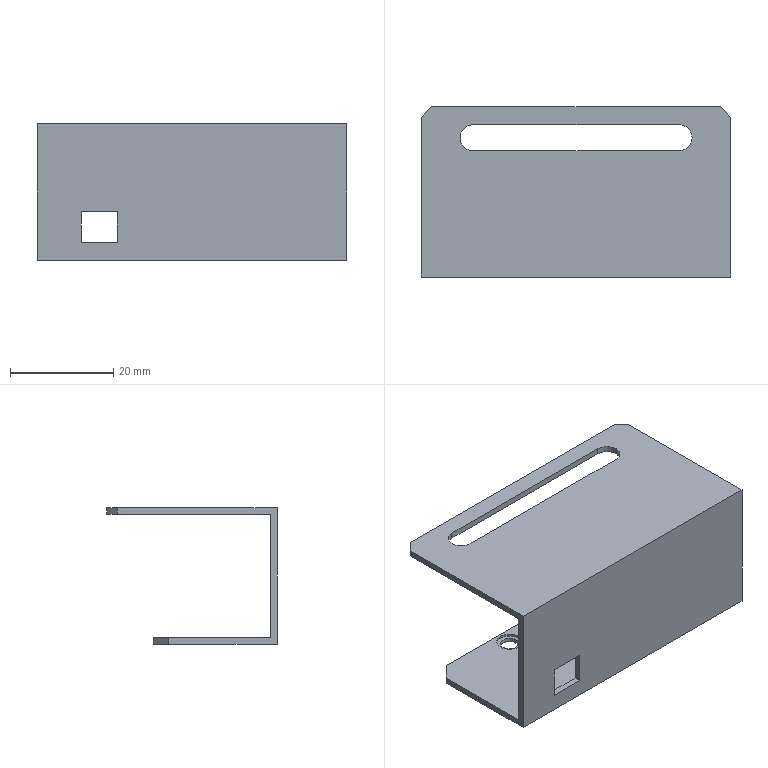Component | SolidWorks | SL010-RightStreamline-1-1_SL010-SensorAssembly-F-1-2_SL010-0ALk-010000-012-2-1-1 | 1 solid | 33 faces | box 60 x 33 x 26.4 mm | volume 5471 mm3 | plane 22 | cylinder 11 | commonest cylinder face diameters 5 x7 3.5 x4 | material 304
build123d program:
from build123d import *

# Parameters (mm, degrees)
SKETCH1_2_W                    = 60
SKETCH1_2_H                    = 33
BOSS_EXTRUDE1_DEPTH            = 1.2
CUT_EXTRUDE1_2_DEPTH           = 35.259
CHAMFER2_SIZE                  = 2
SKETCH6_W                      = 60
SKETCH6_H                      = 1.2
BOSS_EXTRUDE2_DEPTH            = 24
SKETCH7_W                      = 60
SKETCH7_H                      = 24
BOSS_EXTRUDE3_DEPTH            = 1.2
CHAMFER3_SIZE                  = 3
F_3_5_3_5_DIAMETER_HOLE1_D     = 3.5
F_3_5_3_5_DIAMETER_HOLE1_DEPTH = 1.2
SKETCH1_W                      = 7
SKETCH1_H                      = 6
CUT_EXTRUDE1_DEPTH             = 52.071
SKETCH2_R                      = 2.5
CUT_EXTRUDE2_DEPTH             = 0.4


with BuildPart() as part:
    # Sketch1_2 → Boss-Extrude1 (new body)
    with BuildSketch(Plane.XY):
        Rectangle(SKETCH1_2_W, SKETCH1_2_H)
    extrude(amount=BOSS_EXTRUDE1_DEPTH)

    # Sketch2_2 → Cut-Extrude1_2 (cut, through all)
    with BuildSketch(Plane(origin=(0, 0, 0), x_dir=(-1, 0, 0), z_dir=(0, 0, -1))):
        with BuildLine():
            Line((-20, 13), (10, 13))
            ThreePointArc((10, 13), (12.5, 10.5), (10, 8))
            Line((10, 8), (-20, 8))
            ThreePointArc((-20, 8), (-22.5, 10.5), (-20, 13))
        make_face()
    cut_extrude1_2 = extrude(amount=-CUT_EXTRUDE1_2_DEPTH, mode=Mode.SUBTRACT)

    # Mirror1: Cut-Extrude1_2 across plane
    add(cut_extrude1_2.mirror(Plane(origin=(0, 0, 0), x_dir=(0, 0, 1), z_dir=(1, 0, 0))), mode=Mode.SUBTRACT)

    # Chamfer2
    chamfer2_edges = [part.edges().sort_by_distance(p)[0] for p in [
        (-30, 16.5, 0.6),
        (30, 16.5, 0.6),
    ]]
    chamfer(chamfer2_edges, length=CHAMFER2_SIZE)

    # Sketch6 → Boss-Extrude2 (add)
    with BuildSketch(Plane.XY.offset(1.2)):
        with Locations((0, -15.9)):
            Rectangle(SKETCH6_W, SKETCH6_H)
    extrude(amount=BOSS_EXTRUDE2_DEPTH)

    # Sketch7 → Boss-Extrude3 (add)
    with BuildSketch(Plane.XY.offset(25.2)):
        with Locations((0, -4.5)):
            Rectangle(SKETCH7_W, SKETCH7_H)
    extrude(amount=BOSS_EXTRUDE3_DEPTH)

    # Chamfer3
    chamfer3_edges = [part.edges().sort_by_distance(p)[0] for p in [
        (-30, 7.5, 25.8),
        (30, 7.5, 25.8),
    ]]
    chamfer(chamfer3_edges, length=CHAMFER3_SIZE)

    # 3.5 _3.5_ Diameter Hole1
    with Locations(Plane.XY.offset(26.4)):
        with Locations((12.7, 4.5), (-12.7, 4.5)):
            Hole(F_3_5_3_5_DIAMETER_HOLE1_D / 2, depth=F_3_5_3_5_DIAMETER_HOLE1_DEPTH)

    # Sketch1 → Cut-Extrude1 (cut, through all)
    with BuildSketch(Plane(origin=(0, -15.3, 0), x_dir=(1, 0, 0), z_dir=(0, 1, 0))):
        with Locations((18, -20)):
            Rectangle(SKETCH1_W, SKETCH1_H)
    extrude(amount=-CUT_EXTRUDE1_DEPTH, mode=Mode.SUBTRACT)

    # Sketch2 → Cut-Extrude2 (cut)
    with BuildSketch(Plane(origin=(0, 0, 25.2), x_dir=(-1, 0, 0), z_dir=(0, 0, -1))):
        with Locations((-12.7, 4.5)):
            Circle(SKETCH2_R)
        with Locations((12.7, 4.5)):
            Circle(SKETCH2_R)
    extrude(amount=-CUT_EXTRUDE2_DEPTH, mode=Mode.SUBTRACT)


solid = part.part

# Placed as in the assembly
solid = solid.moved(Location((355, -159.904, -331.035), (-180, 0, 180)))
STEP:
#1=COLOUR_RGB('',0.7922,0.8196,0.9333);
#2=FILL_AREA_STYLE_COLOUR('',#1);
#3=FILL_AREA_STYLE('',(#2));
#4=SURFACE_STYLE_FILL_AREA(#3);
#5=SURFACE_SIDE_STYLE('',(#4));
#6=SURFACE_STYLE_USAGE(.BOTH.,#5);
#7=PRESENTATION_STYLE_ASSIGNMENT((#6));
#8=CARTESIAN_POINT('',(14.378,-6.118,-14.041));
#9=VERTEX_POINT('',#8);
#10=CARTESIAN_POINT('',(14.575,-6.118,-14.041));
#11=VERTEX_POINT('',#10);
#12=CARTESIAN_POINT('',(14.476,-6.118,-14.041));
#13=DIRECTION('',(0.,0.,1.));
#14=DIRECTION('',(1.,0.,0.));
#15=AXIS2_PLACEMENT_3D('',#12,#13,#14);
#16=CIRCLE('',#15,0.09843);
#17=EDGE_CURVE('',#9,#11,#16,.T.);
#18=ORIENTED_EDGE('',*,*,#17,.F.);
#19=CARTESIAN_POINT('',(14.378,-6.118,-14.025));
#20=VERTEX_POINT('',#19);
#21=CARTESIAN_POINT('',(14.378,-6.118,-14.041));
#22=DIRECTION('',(0.,0.,1.));
#23=VECTOR('',#22,39.37);
#24=LINE('',#21,#23);
#25=EDGE_CURVE('',#9,#20,#24,.T.);
#26=ORIENTED_EDGE('',*,*,#25,.T.);
#27=CARTESIAN_POINT('',(14.575,-6.118,-14.025));
#28=VERTEX_POINT('',#27);
#29=CARTESIAN_POINT('',(14.476,-6.118,-14.025));
#30=DIRECTION('',(0.,0.,1.));
#31=DIRECTION('',(1.,0.,0.));
#32=AXIS2_PLACEMENT_3D('',#29,#30,#31);
#33=CIRCLE('',#32,0.09843);
#34=EDGE_CURVE('',#20,#28,#33,.T.);
#35=ORIENTED_EDGE('',*,*,#34,.T.);
#36=CARTESIAN_POINT('',(14.575,-6.118,-14.041));
#37=DIRECTION('',(0.,0.,1.));
#38=VECTOR('',#37,39.37);
#39=LINE('',#36,#38);
#40=EDGE_CURVE('',#11,#28,#39,.T.);
#41=ORIENTED_EDGE('',*,*,#40,.F.);
#42=EDGE_LOOP('',(#18,#26,#35,#41));
#43=FACE_OUTER_BOUND('',#42,.T.);
#44=CARTESIAN_POINT('',(14.476,-6.118,-14.041));
#45=DIRECTION('',(0.,0.,1.));
#46=DIRECTION('',(1.,0.,0.));
#47=AXIS2_PLACEMENT_3D('',#44,#45,#46);
#48=CYLINDRICAL_SURFACE('',#47,0.09843);
#49=ADVANCED_FACE('',(#43),#48,.F.);
#50=CARTESIAN_POINT('',(13.378,-6.118,-14.041));
#51=VERTEX_POINT('',#50);
#52=CARTESIAN_POINT('',(13.575,-6.118,-14.041));
#53=VERTEX_POINT('',#52);
#54=CARTESIAN_POINT('',(13.476,-6.118,-14.041));
#55=DIRECTION('',(0.,0.,1.));
#56=DIRECTION('',(1.,0.,0.));
#57=AXIS2_PLACEMENT_3D('',#54,#55,#56);
#58=CIRCLE('',#57,0.09843);
#59=EDGE_CURVE('',#51,#53,#58,.T.);
#60=ORIENTED_EDGE('',*,*,#59,.F.);
#61=CARTESIAN_POINT('',(13.378,-6.118,-14.025));
#62=VERTEX_POINT('',#61);
#63=CARTESIAN_POINT('',(13.378,-6.118,-14.041));
#64=DIRECTION('',(0.,0.,1.));
#65=VECTOR('',#64,39.37);
#66=LINE('',#63,#65);
#67=EDGE_CURVE('',#51,#62,#66,.T.);
#68=ORIENTED_EDGE('',*,*,#67,.T.);
#69=CARTESIAN_POINT('',(13.575,-6.118,-14.025));
#70=VERTEX_POINT('',#69);
#71=CARTESIAN_POINT('',(13.476,-6.118,-14.025));
#72=DIRECTION('',(0.,0.,1.));
#73=DIRECTION('',(1.,0.,0.));
#74=AXIS2_PLACEMENT_3D('',#71,#72,#73);
#75=CIRCLE('',#74,0.09843);
#76=EDGE_CURVE('',#62,#70,#75,.T.);
#77=ORIENTED_EDGE('',*,*,#76,.T.);
#78=CARTESIAN_POINT('',(13.575,-6.118,-14.041));
#79=DIRECTION('',(0.,0.,1.));
#80=VECTOR('',#79,39.37);
#81=LINE('',#78,#80);
#82=EDGE_CURVE('',#53,#70,#81,.T.);
#83=ORIENTED_EDGE('',*,*,#82,.F.);
#84=EDGE_LOOP('',(#60,#68,#77,#83));
#85=FACE_OUTER_BOUND('',#84,.T.);
#86=CARTESIAN_POINT('',(13.476,-6.118,-14.041));
#87=DIRECTION('',(0.,0.,1.));
#88=DIRECTION('',(1.,0.,0.));
#89=AXIS2_PLACEMENT_3D('',#86,#87,#88);
#90=CYLINDRICAL_SURFACE('',#89,0.09843);
#91=ADVANCED_FACE('',(#85),#90,.F.);
#92=CARTESIAN_POINT('',(14.764,-5.784,-13.08));
#93=VERTEX_POINT('',#92);
#94=CARTESIAN_POINT('',(14.862,-5.882,-13.08));
#95=VERTEX_POINT('',#94);
#96=CARTESIAN_POINT('',(14.764,-5.882,-13.08));
#97=DIRECTION('',(-0.,-0.,-1.));
#98=DIRECTION('',(-1.,0.,0.));
#99=AXIS2_PLACEMENT_3D('',#96,#97,#98);
#100=CIRCLE('',#99,0.09843);
#101=EDGE_CURVE('',#93,#95,#100,.T.);
#102=ORIENTED_EDGE('',*,*,#101,.T.);
#103=CARTESIAN_POINT('',(14.862,-5.882,-13.033));
#104=VERTEX_POINT('',#103);
#105=CARTESIAN_POINT('',(14.862,-5.882,-13.08));
#106=DIRECTION('',(0.,0.,1.));
#107=VECTOR('',#106,39.37);
#108=LINE('',#105,#107);
#109=EDGE_CURVE('',#95,#104,#108,.T.);
#110=ORIENTED_EDGE('',*,*,#109,.T.);
#111=CARTESIAN_POINT('',(14.764,-5.784,-13.033));
#112=VERTEX_POINT('',#111);
#113=CARTESIAN_POINT('',(14.764,-5.882,-13.033));
#114=DIRECTION('',(-0.,-0.,-1.));
#115=DIRECTION('',(-1.,0.,0.));
#116=AXIS2_PLACEMENT_3D('',#113,#114,#115);
#117=CIRCLE('',#116,0.09843);
#118=EDGE_CURVE('',#112,#104,#117,.T.);
#119=ORIENTED_EDGE('',*,*,#118,.F.);
#120=CARTESIAN_POINT('',(14.764,-5.784,-13.08));
#121=DIRECTION('',(0.,0.,1.));
#122=VECTOR('',#121,39.37);
#123=LINE('',#120,#122);
#124=EDGE_CURVE('',#93,#112,#123,.T.);
#125=ORIENTED_EDGE('',*,*,#124,.F.);
#126=EDGE_LOOP('',(#102,#110,#119,#125));
#127=FACE_OUTER_BOUND('',#126,.T.);
#128=CARTESIAN_POINT('',(14.764,-5.882,-13.08));
#129=DIRECTION('',(0.,0.,1.));
#130=DIRECTION('',(1.,0.,0.));
#131=AXIS2_PLACEMENT_3D('',#128,#129,#130);
#132=CYLINDRICAL_SURFACE('',#131,0.09843);
#133=ADVANCED_FACE('',(#127),#132,.F.);
#134=CARTESIAN_POINT('',(13.545,-6.118,-14.041));
#135=VERTEX_POINT('',#134);
#136=CARTESIAN_POINT('',(13.407,-6.118,-14.041));
#137=VERTEX_POINT('',#136);
#138=CARTESIAN_POINT('',(13.476,-6.118,-14.041));
#139=DIRECTION('',(-0.,-0.,-1.));
#140=DIRECTION('',(1.,0.,0.));
#141=AXIS2_PLACEMENT_3D('',#138,#139,#140);
#142=CIRCLE('',#141,0.0689);
#143=EDGE_CURVE('',#135,#137,#142,.T.);
#144=ORIENTED_EDGE('',*,*,#143,.F.);
#145=CARTESIAN_POINT('',(13.545,-6.118,-14.072));
#146=VERTEX_POINT('',#145);
#147=CARTESIAN_POINT('',(13.545,-6.118,-14.072));
#148=DIRECTION('',(-0.,-0.,-1.));
#149=VECTOR('',#148,39.37);
#150=LINE('',#147,#149);
#151=EDGE_CURVE('',#135,#146,#150,.T.);
#152=ORIENTED_EDGE('',*,*,#151,.T.);
#153=CARTESIAN_POINT('',(13.407,-6.118,-14.072));
#154=VERTEX_POINT('',#153);
#155=CARTESIAN_POINT('',(13.476,-6.118,-14.072));
#156=DIRECTION('',(-0.,-0.,-1.));
#157=DIRECTION('',(-1.,0.,0.));
#158=AXIS2_PLACEMENT_3D('',#155,#156,#157);
#159=CIRCLE('',#158,0.0689);
#160=EDGE_CURVE('',#146,#154,#159,.T.);
#161=ORIENTED_EDGE('',*,*,#160,.T.);
#162=CARTESIAN_POINT('',(13.407,-6.118,-14.072));
#163=DIRECTION('',(-0.,-0.,-1.));
#164=VECTOR('',#163,39.37);
#165=LINE('',#162,#164);
#166=EDGE_CURVE('',#137,#154,#165,.T.);
#167=ORIENTED_EDGE('',*,*,#166,.F.);
#168=EDGE_LOOP('',(#144,#152,#161,#167));
#169=FACE_OUTER_BOUND('',#168,.T.);
#170=CARTESIAN_POINT('',(13.476,-6.118,-14.072));
#171=DIRECTION('',(-0.,-0.,-1.));
#172=DIRECTION('',(-1.,0.,0.));
#173=AXIS2_PLACEMENT_3D('',#170,#171,#172);
#174=CYLINDRICAL_SURFACE('',#173,0.0689);
#175=ADVANCED_FACE('',(#169),#174,.F.);
#176=CARTESIAN_POINT('',(14.545,-6.118,-14.041));
#177=VERTEX_POINT('',#176);
#178=CARTESIAN_POINT('',(14.407,-6.118,-14.041));
#179=VERTEX_POINT('',#178);
#180=CARTESIAN_POINT('',(14.476,-6.118,-14.041));
#181=DIRECTION('',(-0.,-0.,-1.));
#182=DIRECTION('',(1.,0.,0.));
#183=AXIS2_PLACEMENT_3D('',#180,#181,#182);
#184=CIRCLE('',#183,0.0689);
#185=EDGE_CURVE('',#177,#179,#184,.T.);
#186=ORIENTED_EDGE('',*,*,#185,.F.);
#187=CARTESIAN_POINT('',(14.545,-6.118,-14.072));
#188=VERTEX_POINT('',#187);
#189=CARTESIAN_POINT('',(14.545,-6.118,-14.072));
#190=DIRECTION('',(-0.,-0.,-1.));
#191=VECTOR('',#190,39.37);
#192=LINE('',#189,#191);
#193=EDGE_CURVE('',#177,#188,#192,.T.);
#194=ORIENTED_EDGE('',*,*,#193,.T.);
#195=CARTESIAN_POINT('',(14.407,-6.118,-14.072));
#196=VERTEX_POINT('',#195);
#197=CARTESIAN_POINT('',(14.476,-6.118,-14.072));
#198=DIRECTION('',(-0.,-0.,-1.));
#199=DIRECTION('',(-1.,0.,0.));
#200=AXIS2_PLACEMENT_3D('',#197,#198,#199);
#201=CIRCLE('',#200,0.0689);
#202=EDGE_CURVE('',#188,#196,#201,.T.);
#203=ORIENTED_EDGE('',*,*,#202,.T.);
#204=CARTESIAN_POINT('',(14.407,-6.118,-14.072));
#205=DIRECTION('',(-0.,-0.,-1.));
#206=VECTOR('',#205,39.37);
#207=LINE('',#204,#206);
#208=EDGE_CURVE('',#179,#196,#207,.T.);
#209=ORIENTED_EDGE('',*,*,#208,.F.);
#210=EDGE_LOOP('',(#186,#194,#203,#209));
#211=FACE_OUTER_BOUND('',#210,.T.);
#212=CARTESIAN_POINT('',(14.476,-6.118,-14.072));
#213=DIRECTION('',(-0.,-0.,-1.));
#214=DIRECTION('',(-1.,0.,0.));
#215=AXIS2_PLACEMENT_3D('',#212,#213,#214);
#216=CYLINDRICAL_SURFACE('',#215,0.0689);
#217=ADVANCED_FACE('',(#211),#216,.F.);
#218=ORIENTED_EDGE('',*,*,#193,.F.);
#219=CARTESIAN_POINT('',(14.476,-6.118,-14.041));
#220=DIRECTION('',(-0.,-0.,-1.));
#221=DIRECTION('',(1.,0.,0.));
#222=AXIS2_PLACEMENT_3D('',#219,#220,#221);
#223=CIRCLE('',#222,0.0689);
#224=EDGE_CURVE('',#179,#177,#223,.T.);
#225=ORIENTED_EDGE('',*,*,#224,.F.);
#226=ORIENTED_EDGE('',*,*,#208,.T.);
#227=CARTESIAN_POINT('',(14.476,-6.118,-14.072));
#228=DIRECTION('',(-0.,-0.,-1.));
#229=DIRECTION('',(-1.,0.,0.));
#230=AXIS2_PLACEMENT_3D('',#227,#228,#229);
#231=CIRCLE('',#230,0.0689);
#232=EDGE_CURVE('',#196,#188,#231,.T.);
#233=ORIENTED_EDGE('',*,*,#232,.T.);
#234=EDGE_LOOP('',(#218,#225,#226,#233));
#235=FACE_OUTER_BOUND('',#234,.T.);
#236=CARTESIAN_POINT('',(14.476,-6.118,-14.072));
#237=DIRECTION('',(-0.,-0.,-1.));
#238=DIRECTION('',(-1.,0.,0.));
#239=AXIS2_PLACEMENT_3D('',#236,#237,#238);
#240=CYLINDRICAL_SURFACE('',#239,0.0689);
#241=ADVANCED_FACE('',(#235),#240,.F.);
#242=ORIENTED_EDGE('',*,*,#151,.F.);
#243=CARTESIAN_POINT('',(13.476,-6.118,-14.041));
#244=DIRECTION('',(-0.,-0.,-1.));
#245=DIRECTION('',(1.,0.,0.));
#246=AXIS2_PLACEMENT_3D('',#243,#244,#245);
#247=CIRCLE('',#246,0.0689);
#248=EDGE_CURVE('',#137,#135,#247,.T.);
#249=ORIENTED_EDGE('',*,*,#248,.F.);
#250=ORIENTED_EDGE('',*,*,#166,.T.);
#251=CARTESIAN_POINT('',(13.476,-6.118,-14.072));
#252=DIRECTION('',(-0.,-0.,-1.));
#253=DIRECTION('',(-1.,0.,0.));
#254=AXIS2_PLACEMENT_3D('',#251,#252,#253);
#255=CIRCLE('',#254,0.0689);
#256=EDGE_CURVE('',#154,#146,#255,.T.);
#257=ORIENTED_EDGE('',*,*,#256,.T.);
#258=EDGE_LOOP('',(#242,#249,#250,#257));
#259=FACE_OUTER_BOUND('',#258,.T.);
#260=CARTESIAN_POINT('',(13.476,-6.118,-14.072));
#261=DIRECTION('',(-0.,-0.,-1.));
#262=DIRECTION('',(-1.,0.,0.));
#263=AXIS2_PLACEMENT_3D('',#260,#261,#262);
#264=CYLINDRICAL_SURFACE('',#263,0.0689);
#265=ADVANCED_FACE('',(#259),#264,.F.);
#266=ORIENTED_EDGE('',*,*,#232,.F.);
#267=ORIENTED_EDGE('',*,*,#202,.F.);
#268=EDGE_LOOP('',(#266,#267));
#269=FACE_BOUND('',#268,.T.);
#270=CARTESIAN_POINT('',(12.913,-6.,-14.072));
#271=VERTEX_POINT('',#270);
#272=CARTESIAN_POINT('',(15.039,-6.,-14.072));
#273=VERTEX_POINT('',#272);
#274=CARTESIAN_POINT('',(15.157,-6.,-14.072));
#275=DIRECTION('',(1.,0.,-0.));
#276=VECTOR('',#275,39.37);
#277=LINE('',#274,#276);
#278=EDGE_CURVE('',#271,#273,#277,.T.);
#279=ORIENTED_EDGE('',*,*,#278,.T.);
#280=CARTESIAN_POINT('',(15.157,-6.118,-14.072));
#281=VERTEX_POINT('',#280);
#282=CARTESIAN_POINT('',(15.157,-6.118,-14.072));
#283=DIRECTION('',(0.7071,-0.7071,-0.));
#284=VECTOR('',#283,39.37);
#285=LINE('',#282,#284);
#286=EDGE_CURVE('',#273,#281,#285,.T.);
#287=ORIENTED_EDGE('',*,*,#286,.T.);
#288=CARTESIAN_POINT('',(15.157,-6.945,-14.072));
#289=VERTEX_POINT('',#288);
#290=CARTESIAN_POINT('',(15.157,-6.945,-14.072));
#291=DIRECTION('',(0.,-1.,-0.));
#292=VECTOR('',#291,39.37);
#293=LINE('',#290,#292);
#294=EDGE_CURVE('',#281,#289,#293,.T.);
#295=ORIENTED_EDGE('',*,*,#294,.T.);
#296=CARTESIAN_POINT('',(12.795,-6.945,-14.072));
#297=VERTEX_POINT('',#296);
#298=CARTESIAN_POINT('',(15.157,-6.945,-14.072));
#299=DIRECTION('',(-1.,-0.,0.));
#300=VECTOR('',#299,39.37);
#301=LINE('',#298,#300);
#302=EDGE_CURVE('',#289,#297,#301,.T.);
#303=ORIENTED_EDGE('',*,*,#302,.T.);
#304=CARTESIAN_POINT('',(12.795,-6.118,-14.072));
#305=VERTEX_POINT('',#304);
#306=CARTESIAN_POINT('',(12.795,-6.945,-14.072));
#307=DIRECTION('',(-0.,1.,0.));
#308=VECTOR('',#307,39.37);
#309=LINE('',#306,#308);
#310=EDGE_CURVE('',#297,#305,#309,.T.);
#311=ORIENTED_EDGE('',*,*,#310,.T.);
#312=CARTESIAN_POINT('',(12.913,-6.,-14.072));
#313=DIRECTION('',(0.7071,0.7071,0.));
#314=VECTOR('',#313,39.37);
#315=LINE('',#312,#314);
#316=EDGE_CURVE('',#305,#271,#315,.T.);
#317=ORIENTED_EDGE('',*,*,#316,.T.);
#318=EDGE_LOOP('',(#279,#287,#295,#303,#311,#317));
#319=FACE_OUTER_BOUND('',#318,.T.);
#320=ORIENTED_EDGE('',*,*,#256,.F.);
#321=ORIENTED_EDGE('',*,*,#160,.F.);
#322=EDGE_LOOP('',(#320,#321));
#323=FACE_BOUND('',#322,.T.);
#324=CARTESIAN_POINT('',(13.976,-6.295,-14.072));
#325=DIRECTION('',(0.,0.,1.));
#326=DIRECTION('',(1.,0.,-0.));
#327=AXIS2_PLACEMENT_3D('',#324,#325,#326);
#328=PLANE('',#327);
#329=ADVANCED_FACE('',(#269,#319,#323),#328,.F.);
#330=CARTESIAN_POINT('',(12.795,-6.898,-13.08));
#331=VERTEX_POINT('',#330);
#332=CARTESIAN_POINT('',(15.157,-6.898,-13.08));
#333=VERTEX_POINT('',#332);
#334=CARTESIAN_POINT('',(12.795,-6.898,-13.08));
#335=DIRECTION('',(1.,-0.,-0.));
#336=VECTOR('',#335,39.37);
#337=LINE('',#334,#336);
#338=EDGE_CURVE('',#331,#333,#337,.T.);
#339=ORIENTED_EDGE('',*,*,#338,.F.);
#340=CARTESIAN_POINT('',(12.795,-5.725,-13.08));
#341=VERTEX_POINT('',#340);
#342=CARTESIAN_POINT('',(12.795,-5.646,-13.08));
#343=DIRECTION('',(0.,1.,0.));
#344=VECTOR('',#343,39.37);
#345=LINE('',#342,#344);
#346=EDGE_CURVE('',#331,#341,#345,.T.);
#347=ORIENTED_EDGE('',*,*,#346,.T.);
#348=CARTESIAN_POINT('',(12.874,-5.646,-13.08));
#349=VERTEX_POINT('',#348);
#350=CARTESIAN_POINT('',(13.1,-5.419,-13.08));
#351=DIRECTION('',(0.7071,0.7071,0.));
#352=VECTOR('',#351,39.37);
#353=LINE('',#350,#352);
#354=EDGE_CURVE('',#341,#349,#353,.T.);
#355=ORIENTED_EDGE('',*,*,#354,.T.);
#356=CARTESIAN_POINT('',(15.079,-5.646,-13.08));
#357=VERTEX_POINT('',#356);
#358=CARTESIAN_POINT('',(15.157,-5.646,-13.08));
#359=DIRECTION('',(1.,0.,-0.));
#360=VECTOR('',#359,39.37);
#361=LINE('',#358,#360);
#362=EDGE_CURVE('',#349,#357,#361,.T.);
#363=ORIENTED_EDGE('',*,*,#362,.T.);
#364=CARTESIAN_POINT('',(15.157,-5.725,-13.08));
#365=VERTEX_POINT('',#364);
#366=CARTESIAN_POINT('',(14.852,-5.419,-13.08));
#367=DIRECTION('',(0.7071,-0.7071,-0.));
#368=VECTOR('',#367,39.37);
#369=LINE('',#366,#368);
#370=EDGE_CURVE('',#357,#365,#369,.T.);
#371=ORIENTED_EDGE('',*,*,#370,.T.);
#372=CARTESIAN_POINT('',(15.157,-5.646,-13.08));
#373=DIRECTION('',(-0.,-1.,-0.));
#374=VECTOR('',#373,39.37);
#375=LINE('',#372,#374);
#376=EDGE_CURVE('',#365,#333,#375,.T.);
#377=ORIENTED_EDGE('',*,*,#376,.T.);
#378=EDGE_LOOP('',(#339,#347,#355,#363,#371,#377));
#379=FACE_OUTER_BOUND('',#378,.T.);
#380=CARTESIAN_POINT('',(13.189,-5.98,-13.08));
#381=VERTEX_POINT('',#380);
#382=CARTESIAN_POINT('',(14.764,-5.98,-13.08));
#383=VERTEX_POINT('',#382);
#384=CARTESIAN_POINT('',(13.189,-5.98,-13.08));
#385=DIRECTION('',(1.,0.,-0.));
#386=VECTOR('',#385,39.37);
#387=LINE('',#384,#386);
#388=EDGE_CURVE('',#381,#383,#387,.T.);
#389=ORIENTED_EDGE('',*,*,#388,.T.);
#390=CARTESIAN_POINT('',(14.764,-5.882,-13.08));
#391=DIRECTION('',(-0.,-0.,-1.));
#392=DIRECTION('',(-1.,0.,0.));
#393=AXIS2_PLACEMENT_3D('',#390,#391,#392);
#394=CIRCLE('',#393,0.09843);
#395=EDGE_CURVE('',#95,#383,#394,.T.);
#396=ORIENTED_EDGE('',*,*,#395,.F.);
#397=ORIENTED_EDGE('',*,*,#101,.F.);
#398=CARTESIAN_POINT('',(13.189,-5.784,-13.08));
#399=VERTEX_POINT('',#398);
#400=CARTESIAN_POINT('',(13.189,-5.784,-13.08));
#401=DIRECTION('',(-1.,-0.,0.));
#402=VECTOR('',#401,39.37);
#403=LINE('',#400,#402);
#404=EDGE_CURVE('',#93,#399,#403,.T.);
#405=ORIENTED_EDGE('',*,*,#404,.T.);
#406=CARTESIAN_POINT('',(13.189,-5.882,-13.08));
#407=DIRECTION('',(0.,0.,1.));
#408=DIRECTION('',(1.,0.,0.));
#409=AXIS2_PLACEMENT_3D('',#406,#407,#408);
#410=CIRCLE('',#409,0.09843);
#411=EDGE_CURVE('',#399,#381,#410,.T.);
#412=ORIENTED_EDGE('',*,*,#411,.T.);
#413=EDGE_LOOP('',(#389,#396,#397,#405,#412));
#414=FACE_BOUND('',#413,.T.);
#415=CARTESIAN_POINT('',(13.976,-6.295,-13.08));
#416=DIRECTION('',(-0.,-0.,-1.));
#417=DIRECTION('',(-1.,-0.,0.));
#418=AXIS2_PLACEMENT_3D('',#415,#416,#417);
#419=PLANE('',#418);
#420=ADVANCED_FACE('',(#379,#414),#419,.T.);
#421=CARTESIAN_POINT('',(12.874,-5.646,-13.033));
#422=VERTEX_POINT('',#421);
#423=CARTESIAN_POINT('',(15.079,-5.646,-13.033));
#424=VERTEX_POINT('',#423);
#425=CARTESIAN_POINT('',(15.157,-5.646,-13.033));
#426=DIRECTION('',(1.,0.,-0.));
#427=VECTOR('',#426,39.37);
#428=LINE('',#425,#427);
#429=EDGE_CURVE('',#422,#424,#428,.T.);
#430=ORIENTED_EDGE('',*,*,#429,.F.);
#431=CARTESIAN_POINT('',(12.795,-5.725,-13.033));
#432=VERTEX_POINT('',#431);
#433=CARTESIAN_POINT('',(12.874,-5.646,-13.033));
#434=DIRECTION('',(-0.7071,-0.7071,-0.));
#435=VECTOR('',#434,39.37);
#436=LINE('',#433,#435);
#437=EDGE_CURVE('',#422,#432,#436,.T.);
#438=ORIENTED_EDGE('',*,*,#437,.T.);
#439=CARTESIAN_POINT('',(12.795,-6.945,-13.033));
#440=VERTEX_POINT('',#439);
#441=CARTESIAN_POINT('',(12.795,-5.646,-13.033));
#442=DIRECTION('',(0.,1.,0.));
#443=VECTOR('',#442,39.37);
#444=LINE('',#441,#443);
#445=EDGE_CURVE('',#440,#432,#444,.T.);
#446=ORIENTED_EDGE('',*,*,#445,.F.);
#447=CARTESIAN_POINT('',(15.157,-6.945,-13.033));
#448=VERTEX_POINT('',#447);
#449=CARTESIAN_POINT('',(15.157,-6.945,-13.033));
#450=DIRECTION('',(-1.,-0.,0.));
#451=VECTOR('',#450,39.37);
#452=LINE('',#449,#451);
#453=EDGE_CURVE('',#448,#440,#452,.T.);
#454=ORIENTED_EDGE('',*,*,#453,.F.);
#455=CARTESIAN_POINT('',(15.157,-5.725,-13.033));
#456=VERTEX_POINT('',#455);
#457=CARTESIAN_POINT('',(15.157,-5.646,-13.033));
#458=DIRECTION('',(-0.,-1.,-0.));
#459=VECTOR('',#458,39.37);
#460=LINE('',#457,#459);
#461=EDGE_CURVE('',#456,#448,#460,.T.);
#462=ORIENTED_EDGE('',*,*,#461,.F.);
#463=CARTESIAN_POINT('',(15.157,-5.725,-13.033));
#464=DIRECTION('',(-0.7071,0.7071,0.));
#465=VECTOR('',#464,39.37);
#466=LINE('',#463,#465);
#467=EDGE_CURVE('',#456,#424,#466,.T.);
#468=ORIENTED_EDGE('',*,*,#467,.T.);
#469=EDGE_LOOP('',(#430,#438,#446,#454,#462,#468));
#470=FACE_OUTER_BOUND('',#469,.T.);
#471=ORIENTED_EDGE('',*,*,#118,.T.);
#472=CARTESIAN_POINT('',(14.764,-5.98,-13.033));
#473=VERTEX_POINT('',#472);
#474=CARTESIAN_POINT('',(14.764,-5.882,-13.033));
#475=DIRECTION('',(-0.,-0.,-1.));
#476=DIRECTION('',(-1.,0.,0.));
#477=AXIS2_PLACEMENT_3D('',#474,#475,#476);
#478=CIRCLE('',#477,0.09843);
#479=EDGE_CURVE('',#104,#473,#478,.T.);
#480=ORIENTED_EDGE('',*,*,#479,.T.);
#481=CARTESIAN_POINT('',(13.189,-5.98,-13.033));
#482=VERTEX_POINT('',#481);
#483=CARTESIAN_POINT('',(13.189,-5.98,-13.033));
#484=DIRECTION('',(1.,0.,-0.));
#485=VECTOR('',#484,39.37);
#486=LINE('',#483,#485);
#487=EDGE_CURVE('',#482,#473,#486,.T.);
#488=ORIENTED_EDGE('',*,*,#487,.F.);
#489=CARTESIAN_POINT('',(13.189,-5.784,-13.033));
#490=VERTEX_POINT('',#489);
#491=CARTESIAN_POINT('',(13.189,-5.882,-13.033));
#492=DIRECTION('',(0.,0.,1.));
#493=DIRECTION('',(1.,0.,0.));
#494=AXIS2_PLACEMENT_3D('',#491,#492,#493);
#495=CIRCLE('',#494,0.09843);
#496=EDGE_CURVE('',#490,#482,#495,.T.);
#497=ORIENTED_EDGE('',*,*,#496,.F.);
#498=CARTESIAN_POINT('',(13.189,-5.784,-13.033));
#499=DIRECTION('',(-1.,-0.,0.));
#500=VECTOR('',#499,39.37);
#501=LINE('',#498,#500);
#502=EDGE_CURVE('',#112,#490,#501,.T.);
#503=ORIENTED_EDGE('',*,*,#502,.F.);
#504=EDGE_LOOP('',(#471,#480,#488,#497,#503));
#505=FACE_BOUND('',#504,.T.);
#506=CARTESIAN_POINT('',(13.976,-6.295,-13.033));
#507=DIRECTION('',(-0.,-0.,-1.));
#508=DIRECTION('',(-1.,-0.,0.));
#509=AXIS2_PLACEMENT_3D('',#506,#507,#508);
#510=PLANE('',#509);
#511=ADVANCED_FACE('',(#470,#505),#510,.F.);
#512=CARTESIAN_POINT('',(12.795,-6.898,-14.025));
#513=VERTEX_POINT('',#512);
#514=CARTESIAN_POINT('',(12.795,-6.118,-14.025));
#515=VERTEX_POINT('',#514);
#516=CARTESIAN_POINT('',(12.795,-6.945,-14.025));
#517=DIRECTION('',(-0.,1.,0.));
#518=VECTOR('',#517,39.37);
#519=LINE('',#516,#518);
#520=EDGE_CURVE('',#513,#515,#519,.T.);
#521=ORIENTED_EDGE('',*,*,#520,.T.);
#522=CARTESIAN_POINT('',(12.795,-6.118,-13.08));
#523=DIRECTION('',(-0.,-0.,-1.));
#524=VECTOR('',#523,39.37);
#525=LINE('',#522,#524);
#526=EDGE_CURVE('',#515,#305,#525,.T.);
#527=ORIENTED_EDGE('',*,*,#526,.T.);
#528=ORIENTED_EDGE('',*,*,#310,.F.);
#529=CARTESIAN_POINT('',(12.795,-6.945,-13.08));
#530=DIRECTION('',(0.,0.,1.));
#531=VECTOR('',#530,39.37);
#532=LINE('',#529,#531);
#533=EDGE_CURVE('',#297,#440,#532,.T.);
#534=ORIENTED_EDGE('',*,*,#533,.T.);
#535=ORIENTED_EDGE('',*,*,#445,.T.);
#536=CARTESIAN_POINT('',(12.795,-5.725,-13.08));
#537=DIRECTION('',(-0.,-0.,-1.));
#538=VECTOR('',#537,39.37);
#539=LINE('',#536,#538);
#540=EDGE_CURVE('',#432,#341,#539,.T.);
#541=ORIENTED_EDGE('',*,*,#540,.T.);
#542=ORIENTED_EDGE('',*,*,#346,.F.);
#543=CARTESIAN_POINT('',(12.795,-6.898,-14.025));
#544=DIRECTION('',(0.,0.,1.));
#545=VECTOR('',#544,39.37);
#546=LINE('',#543,#545);
#547=EDGE_CURVE('',#513,#331,#546,.T.);
#548=ORIENTED_EDGE('',*,*,#547,.F.);
#549=EDGE_LOOP('',(#521,#527,#528,#534,#535,#541,#542,#548));
#550=FACE_OUTER_BOUND('',#549,.T.);
#551=CARTESIAN_POINT('',(12.795,-5.646,-13.08));
#552=DIRECTION('',(1.,-0.,-0.));
#553=DIRECTION('',(-0.,-1.,-0.));
#554=AXIS2_PLACEMENT_3D('',#551,#552,#553);
#555=PLANE('',#554);
#556=ADVANCED_FACE('',(#550),#555,.F.);
#557=ORIENTED_EDGE('',*,*,#362,.F.);
#558=CARTESIAN_POINT('',(12.874,-5.646,-13.08));
#559=DIRECTION('',(0.,0.,1.));
#560=VECTOR('',#559,39.37);
#561=LINE('',#558,#560);
#562=EDGE_CURVE('',#349,#422,#561,.T.);
#563=ORIENTED_EDGE('',*,*,#562,.T.);
#564=ORIENTED_EDGE('',*,*,#429,.T.);
#565=CARTESIAN_POINT('',(15.079,-5.646,-13.08));
#566=DIRECTION('',(-0.,-0.,-1.));
#567=VECTOR('',#566,39.37);
#568=LINE('',#565,#567);
#569=EDGE_CURVE('',#424,#357,#568,.T.);
#570=ORIENTED_EDGE('',*,*,#569,.T.);
#571=EDGE_LOOP('',(#557,#563,#564,#570));
#572=FACE_OUTER_BOUND('',#571,.T.);
#573=CARTESIAN_POINT('',(15.157,-5.646,-13.08));
#574=DIRECTION('',(0.,-1.,0.));
#575=DIRECTION('',(0.,0.,1.));
#576=AXIS2_PLACEMENT_3D('',#573,#574,#575);
#577=PLANE('',#576);
#578=ADVANCED_FACE('',(#572),#577,.F.);
#579=ORIENTED_EDGE('',*,*,#294,.F.);
#580=CARTESIAN_POINT('',(15.157,-6.118,-14.025));
#581=VERTEX_POINT('',#580);
#582=CARTESIAN_POINT('',(15.157,-6.118,-13.08));
#583=DIRECTION('',(0.,0.,1.));
#584=VECTOR('',#583,39.37);
#585=LINE('',#582,#584);
#586=EDGE_CURVE('',#281,#581,#585,.T.);
#587=ORIENTED_EDGE('',*,*,#586,.T.);
#588=CARTESIAN_POINT('',(15.157,-6.898,-14.025));
#589=VERTEX_POINT('',#588);
#590=CARTESIAN_POINT('',(15.157,-6.945,-14.025));
#591=DIRECTION('',(0.,-1.,-0.));
#592=VECTOR('',#591,39.37);
#593=LINE('',#590,#592);
#594=EDGE_CURVE('',#581,#589,#593,.T.);
#595=ORIENTED_EDGE('',*,*,#594,.T.);
#596=CARTESIAN_POINT('',(15.157,-6.898,-14.025));
#597=DIRECTION('',(0.,0.,1.));
#598=VECTOR('',#597,39.37);
#599=LINE('',#596,#598);
#600=EDGE_CURVE('',#589,#333,#599,.T.);
#601=ORIENTED_EDGE('',*,*,#600,.T.);
#602=ORIENTED_EDGE('',*,*,#376,.F.);
#603=CARTESIAN_POINT('',(15.157,-5.725,-13.08));
#604=DIRECTION('',(0.,0.,1.));
#605=VECTOR('',#604,39.37);
#606=LINE('',#603,#605);
#607=EDGE_CURVE('',#365,#456,#606,.T.);
#608=ORIENTED_EDGE('',*,*,#607,.T.);
#609=ORIENTED_EDGE('',*,*,#461,.T.);
#610=CARTESIAN_POINT('',(15.157,-6.945,-13.08));
#611=DIRECTION('',(0.,0.,1.));
#612=VECTOR('',#611,39.37);
#613=LINE('',#610,#612);
#614=EDGE_CURVE('',#289,#448,#613,.T.);
#615=ORIENTED_EDGE('',*,*,#614,.F.);
#616=EDGE_LOOP('',(#579,#587,#595,#601,#602,#608,#609,#615));
#617=FACE_OUTER_BOUND('',#616,.T.);
#618=CARTESIAN_POINT('',(15.157,-5.646,-13.08));
#619=DIRECTION('',(-1.,0.,0.));
#620=DIRECTION('',(0.,1.,0.));
#621=AXIS2_PLACEMENT_3D('',#618,#619,#620);
#622=PLANE('',#621);
#623=ADVANCED_FACE('',(#617),#622,.F.);
#624=CARTESIAN_POINT('',(13.406,-6.945,-13.938));
#625=VERTEX_POINT('',#624);
#626=CARTESIAN_POINT('',(13.13,-6.945,-13.938));
#627=VERTEX_POINT('',#626);
#628=CARTESIAN_POINT('',(13.13,-6.945,-13.938));
#629=DIRECTION('',(-1.,-0.,0.));
#630=VECTOR('',#629,39.37);
#631=LINE('',#628,#630);
#632=EDGE_CURVE('',#625,#627,#631,.T.);
#633=ORIENTED_EDGE('',*,*,#632,.T.);
#634=CARTESIAN_POINT('',(13.13,-6.945,-13.702));
#635=VERTEX_POINT('',#634);
#636=CARTESIAN_POINT('',(13.13,-6.945,-13.938));
#637=DIRECTION('',(0.,0.,1.));
#638=VECTOR('',#637,39.37);
#639=LINE('',#636,#638);
#640=EDGE_CURVE('',#627,#635,#639,.T.);
#641=ORIENTED_EDGE('',*,*,#640,.T.);
#642=CARTESIAN_POINT('',(13.406,-6.945,-13.702));
#643=VERTEX_POINT('',#642);
#644=CARTESIAN_POINT('',(13.13,-6.945,-13.702));
#645=DIRECTION('',(1.,0.,-0.));
#646=VECTOR('',#645,39.37);
#647=LINE('',#644,#646);
#648=EDGE_CURVE('',#635,#643,#647,.T.);
#649=ORIENTED_EDGE('',*,*,#648,.T.);
#650=CARTESIAN_POINT('',(13.406,-6.945,-13.938));
#651=DIRECTION('',(-0.,-0.,-1.));
#652=VECTOR('',#651,39.37);
#653=LINE('',#650,#652);
#654=EDGE_CURVE('',#643,#625,#653,.T.);
#655=ORIENTED_EDGE('',*,*,#654,.T.);
#656=EDGE_LOOP('',(#633,#641,#649,#655));
#657=FACE_BOUND('',#656,.T.);
#658=ORIENTED_EDGE('',*,*,#453,.T.);
#659=ORIENTED_EDGE('',*,*,#533,.F.);
#660=ORIENTED_EDGE('',*,*,#302,.F.);
#661=ORIENTED_EDGE('',*,*,#614,.T.);
#662=EDGE_LOOP('',(#658,#659,#660,#661));
#663=FACE_OUTER_BOUND('',#662,.T.);
#664=CARTESIAN_POINT('',(15.157,-6.945,-13.08));
#665=DIRECTION('',(-0.,1.,-0.));
#666=DIRECTION('',(-0.,-0.,-1.));
#667=AXIS2_PLACEMENT_3D('',#664,#665,#666);
#668=PLANE('',#667);
#669=ADVANCED_FACE('',(#657,#663),#668,.F.);
#670=ORIENTED_EDGE('',*,*,#496,.T.);
#671=CARTESIAN_POINT('',(13.189,-5.98,-13.08));
#672=DIRECTION('',(0.,0.,1.));
#673=VECTOR('',#672,39.37);
#674=LINE('',#671,#673);
#675=EDGE_CURVE('',#381,#482,#674,.T.);
#676=ORIENTED_EDGE('',*,*,#675,.F.);
#677=ORIENTED_EDGE('',*,*,#411,.F.);
#678=CARTESIAN_POINT('',(13.189,-5.784,-13.08));
#679=DIRECTION('',(0.,0.,1.));
#680=VECTOR('',#679,39.37);
#681=LINE('',#678,#680);
#682=EDGE_CURVE('',#399,#490,#681,.T.);
#683=ORIENTED_EDGE('',*,*,#682,.T.);
#684=EDGE_LOOP('',(#670,#676,#677,#683));
#685=FACE_OUTER_BOUND('',#684,.T.);
#686=CARTESIAN_POINT('',(13.189,-5.882,-13.08));
#687=DIRECTION('',(0.,0.,1.));
#688=DIRECTION('',(1.,0.,0.));
#689=AXIS2_PLACEMENT_3D('',#686,#687,#688);
#690=CYLINDRICAL_SURFACE('',#689,0.09843);
#691=ADVANCED_FACE('',(#685),#690,.F.);
#692=ORIENTED_EDGE('',*,*,#502,.T.);
#693=ORIENTED_EDGE('',*,*,#682,.F.);
#694=ORIENTED_EDGE('',*,*,#404,.F.);
#695=ORIENTED_EDGE('',*,*,#124,.T.);
#696=EDGE_LOOP('',(#692,#693,#694,#695));
#697=FACE_OUTER_BOUND('',#696,.T.);
#698=CARTESIAN_POINT('',(13.189,-5.784,-13.08));
#699=DIRECTION('',(-0.,1.,-0.));
#700=DIRECTION('',(-0.,-0.,-1.));
#701=AXIS2_PLACEMENT_3D('',#698,#699,#700);
#702=PLANE('',#701);
#703=ADVANCED_FACE('',(#697),#702,.F.);
#704=ORIENTED_EDGE('',*,*,#487,.T.);
#705=CARTESIAN_POINT('',(14.764,-5.98,-13.08));
#706=DIRECTION('',(0.,0.,1.));
#707=VECTOR('',#706,39.37);
#708=LINE('',#705,#707);
#709=EDGE_CURVE('',#383,#473,#708,.T.);
#710=ORIENTED_EDGE('',*,*,#709,.F.);
#711=ORIENTED_EDGE('',*,*,#388,.F.);
#712=ORIENTED_EDGE('',*,*,#675,.T.);
#713=EDGE_LOOP('',(#704,#710,#711,#712));
#714=FACE_OUTER_BOUND('',#713,.T.);
#715=CARTESIAN_POINT('',(13.189,-5.98,-13.08));
#716=DIRECTION('',(0.,-1.,0.));
#717=DIRECTION('',(0.,0.,1.));
#718=AXIS2_PLACEMENT_3D('',#715,#716,#717);
#719=PLANE('',#718);
#720=ADVANCED_FACE('',(#714),#719,.F.);
#721=ORIENTED_EDGE('',*,*,#109,.F.);
#722=ORIENTED_EDGE('',*,*,#395,.T.);
#723=ORIENTED_EDGE('',*,*,#709,.T.);
#724=ORIENTED_EDGE('',*,*,#479,.F.);
#725=EDGE_LOOP('',(#721,#722,#723,#724));
#726=FACE_OUTER_BOUND('',#725,.T.);
#727=CARTESIAN_POINT('',(14.764,-5.882,-13.08));
#728=DIRECTION('',(0.,0.,1.));
#729=DIRECTION('',(1.,0.,0.));
#730=AXIS2_PLACEMENT_3D('',#727,#728,#729);
#731=CYLINDRICAL_SURFACE('',#730,0.09843);
#732=ADVANCED_FACE('',(#726),#731,.F.);
#733=ORIENTED_EDGE('',*,*,#354,.F.);
#734=ORIENTED_EDGE('',*,*,#540,.F.);
#735=ORIENTED_EDGE('',*,*,#437,.F.);
#736=ORIENTED_EDGE('',*,*,#562,.F.);
#737=EDGE_LOOP('',(#733,#734,#735,#736));
#738=FACE_OUTER_BOUND('',#737,.T.);
#739=CARTESIAN_POINT('',(12.874,-5.646,-13.08));
#740=DIRECTION('',(0.7071,-0.7071,-0.));
#741=DIRECTION('',(0.,0.,1.));
#742=AXIS2_PLACEMENT_3D('',#739,#740,#741);
#743=PLANE('',#742);
#744=ADVANCED_FACE('',(#738),#743,.F.);
#745=ORIENTED_EDGE('',*,*,#370,.F.);
#746=ORIENTED_EDGE('',*,*,#569,.F.);
#747=ORIENTED_EDGE('',*,*,#467,.F.);
#748=ORIENTED_EDGE('',*,*,#607,.F.);
#749=EDGE_LOOP('',(#745,#746,#747,#748));
#750=FACE_OUTER_BOUND('',#749,.T.);
#751=CARTESIAN_POINT('',(15.157,-5.725,-13.08));
#752=DIRECTION('',(-0.7071,-0.7071,0.));
#753=DIRECTION('',(0.,0.,1.));
#754=AXIS2_PLACEMENT_3D('',#751,#752,#753);
#755=PLANE('',#754);
#756=ADVANCED_FACE('',(#750),#755,.F.);
#757=CARTESIAN_POINT('',(13.13,-6.898,-13.702));
#758=VERTEX_POINT('',#757);
#759=CARTESIAN_POINT('',(13.406,-6.898,-13.702));
#760=VERTEX_POINT('',#759);
#761=CARTESIAN_POINT('',(13.13,-6.898,-13.702));
#762=DIRECTION('',(1.,0.,-0.));
#763=VECTOR('',#762,39.37);
#764=LINE('',#761,#763);
#765=EDGE_CURVE('',#758,#760,#764,.T.);
#766=ORIENTED_EDGE('',*,*,#765,.F.);
#767=CARTESIAN_POINT('',(13.13,-6.898,-13.938));
#768=VERTEX_POINT('',#767);
#769=CARTESIAN_POINT('',(13.13,-6.898,-13.938));
#770=DIRECTION('',(0.,0.,1.));
#771=VECTOR('',#770,39.37);
#772=LINE('',#769,#771);
#773=EDGE_CURVE('',#768,#758,#772,.T.);
#774=ORIENTED_EDGE('',*,*,#773,.F.);
#775=CARTESIAN_POINT('',(13.406,-6.898,-13.938));
#776=VERTEX_POINT('',#775);
#777=CARTESIAN_POINT('',(13.13,-6.898,-13.938));
#778=DIRECTION('',(-1.,-0.,0.));
#779=VECTOR('',#778,39.37);
#780=LINE('',#777,#779);
#781=EDGE_CURVE('',#776,#768,#780,.T.);
#782=ORIENTED_EDGE('',*,*,#781,.F.);
#783=CARTESIAN_POINT('',(13.406,-6.898,-13.938));
#784=DIRECTION('',(-0.,-0.,-1.));
#785=VECTOR('',#784,39.37);
#786=LINE('',#783,#785);
#787=EDGE_CURVE('',#760,#776,#786,.T.);
#788=ORIENTED_EDGE('',*,*,#787,.F.);
#789=EDGE_LOOP('',(#766,#774,#782,#788));
#790=FACE_BOUND('',#789,.T.);
#791=ORIENTED_EDGE('',*,*,#338,.T.);
#792=ORIENTED_EDGE('',*,*,#600,.F.);
#793=CARTESIAN_POINT('',(12.795,-6.898,-14.025));
#794=DIRECTION('',(1.,-0.,-0.));
#795=VECTOR('',#794,39.37);
#796=LINE('',#793,#795);
#797=EDGE_CURVE('',#513,#589,#796,.T.);
#798=ORIENTED_EDGE('',*,*,#797,.F.);
#799=ORIENTED_EDGE('',*,*,#547,.T.);
#800=EDGE_LOOP('',(#791,#792,#798,#799));
#801=FACE_OUTER_BOUND('',#800,.T.);
#802=CARTESIAN_POINT('',(12.795,-6.898,-14.025));
#803=DIRECTION('',(-0.,-1.,-0.));
#804=DIRECTION('',(-1.,0.,0.));
#805=AXIS2_PLACEMENT_3D('',#802,#803,#804);
#806=PLANE('',#805);
#807=ADVANCED_FACE('',(#790,#801),#806,.F.);
#808=CARTESIAN_POINT('',(12.913,-6.,-14.025));
#809=VERTEX_POINT('',#808);
#810=CARTESIAN_POINT('',(15.039,-6.,-14.025));
#811=VERTEX_POINT('',#810);
#812=CARTESIAN_POINT('',(15.157,-6.,-14.025));
#813=DIRECTION('',(1.,0.,-0.));
#814=VECTOR('',#813,39.37);
#815=LINE('',#812,#814);
#816=EDGE_CURVE('',#809,#811,#815,.T.);
#817=ORIENTED_EDGE('',*,*,#816,.T.);
#818=CARTESIAN_POINT('',(15.039,-6.,-14.072));
#819=DIRECTION('',(-0.,-0.,-1.));
#820=VECTOR('',#819,39.37);
#821=LINE('',#818,#820);
#822=EDGE_CURVE('',#811,#273,#821,.T.);
#823=ORIENTED_EDGE('',*,*,#822,.T.);
#824=ORIENTED_EDGE('',*,*,#278,.F.);
#825=CARTESIAN_POINT('',(12.913,-6.,-14.072));
#826=DIRECTION('',(0.,0.,1.));
#827=VECTOR('',#826,39.37);
#828=LINE('',#825,#827);
#829=EDGE_CURVE('',#271,#809,#828,.T.);
#830=ORIENTED_EDGE('',*,*,#829,.T.);
#831=EDGE_LOOP('',(#817,#823,#824,#830));
#832=FACE_OUTER_BOUND('',#831,.T.);
#833=CARTESIAN_POINT('',(15.157,-6.,-14.072));
#834=DIRECTION('',(0.,-1.,0.));
#835=DIRECTION('',(0.,0.,1.));
#836=AXIS2_PLACEMENT_3D('',#833,#834,#835);
#837=PLANE('',#836);
#838=ADVANCED_FACE('',(#832),#837,.F.);
#839=CARTESIAN_POINT('',(13.476,-6.118,-14.025));
#840=DIRECTION('',(0.,0.,1.));
#841=DIRECTION('',(1.,0.,0.));
#842=AXIS2_PLACEMENT_3D('',#839,#840,#841);
#843=CIRCLE('',#842,0.09843);
#844=EDGE_CURVE('',#70,#62,#843,.T.);
#845=ORIENTED_EDGE('',*,*,#844,.F.);
#846=ORIENTED_EDGE('',*,*,#76,.F.);
#847=EDGE_LOOP('',(#845,#846));
#848=FACE_BOUND('',#847,.T.);
#849=CARTESIAN_POINT('',(14.476,-6.118,-14.025));
#850=DIRECTION('',(0.,0.,1.));
#851=DIRECTION('',(1.,0.,0.));
#852=AXIS2_PLACEMENT_3D('',#849,#850,#851);
#853=CIRCLE('',#852,0.09843);
#854=EDGE_CURVE('',#28,#20,#853,.T.);
#855=ORIENTED_EDGE('',*,*,#854,.F.);
#856=ORIENTED_EDGE('',*,*,#34,.F.);
#857=EDGE_LOOP('',(#855,#856));
#858=FACE_BOUND('',#857,.T.);
#859=ORIENTED_EDGE('',*,*,#594,.F.);
#860=CARTESIAN_POINT('',(14.656,-5.616,-14.025));
#861=DIRECTION('',(-0.7071,0.7071,0.));
#862=VECTOR('',#861,39.37);
#863=LINE('',#860,#862);
#864=EDGE_CURVE('',#581,#811,#863,.T.);
#865=ORIENTED_EDGE('',*,*,#864,.T.);
#866=ORIENTED_EDGE('',*,*,#816,.F.);
#867=CARTESIAN_POINT('',(13.297,-5.616,-14.025));
#868=DIRECTION('',(-0.7071,-0.7071,-0.));
#869=VECTOR('',#868,39.37);
#870=LINE('',#867,#869);
#871=EDGE_CURVE('',#809,#515,#870,.T.);
#872=ORIENTED_EDGE('',*,*,#871,.T.);
#873=ORIENTED_EDGE('',*,*,#520,.F.);
#874=ORIENTED_EDGE('',*,*,#797,.T.);
#875=EDGE_LOOP('',(#859,#865,#866,#872,#873,#874));
#876=FACE_OUTER_BOUND('',#875,.T.);
#877=CARTESIAN_POINT('',(13.976,-6.295,-14.025));
#878=DIRECTION('',(0.,0.,1.));
#879=DIRECTION('',(1.,0.,-0.));
#880=AXIS2_PLACEMENT_3D('',#877,#878,#879);
#881=PLANE('',#880);
#882=ADVANCED_FACE('',(#848,#858,#876),#881,.T.);
#883=ORIENTED_EDGE('',*,*,#286,.F.);
#884=ORIENTED_EDGE('',*,*,#822,.F.);
#885=ORIENTED_EDGE('',*,*,#864,.F.);
#886=ORIENTED_EDGE('',*,*,#586,.F.);
#887=EDGE_LOOP('',(#883,#884,#885,#886));
#888=FACE_OUTER_BOUND('',#887,.T.);
#889=CARTESIAN_POINT('',(15.157,-6.118,-13.08));
#890=DIRECTION('',(-0.7071,-0.7071,0.));
#891=DIRECTION('',(0.,0.,1.));
#892=AXIS2_PLACEMENT_3D('',#889,#890,#891);
#893=PLANE('',#892);
#894=ADVANCED_FACE('',(#888),#893,.F.);
#895=ORIENTED_EDGE('',*,*,#316,.F.);
#896=ORIENTED_EDGE('',*,*,#526,.F.);
#897=ORIENTED_EDGE('',*,*,#871,.F.);
#898=ORIENTED_EDGE('',*,*,#829,.F.);
#899=EDGE_LOOP('',(#895,#896,#897,#898));
#900=FACE_OUTER_BOUND('',#899,.T.);
#901=CARTESIAN_POINT('',(12.913,-6.,-14.072));
#902=DIRECTION('',(0.7071,-0.7071,-0.));
#903=DIRECTION('',(0.,0.,1.));
#904=AXIS2_PLACEMENT_3D('',#901,#902,#903);
#905=PLANE('',#904);
#906=ADVANCED_FACE('',(#900),#905,.F.);
#907=ORIENTED_EDGE('',*,*,#773,.T.);
#908=CARTESIAN_POINT('',(13.13,-6.945,-13.702));
#909=DIRECTION('',(0.,1.,0.));
#910=VECTOR('',#909,39.37);
#911=LINE('',#908,#910);
#912=EDGE_CURVE('',#635,#758,#911,.T.);
#913=ORIENTED_EDGE('',*,*,#912,.F.);
#914=ORIENTED_EDGE('',*,*,#640,.F.);
#915=CARTESIAN_POINT('',(13.13,-6.945,-13.938));
#916=DIRECTION('',(0.,1.,0.));
#917=VECTOR('',#916,39.37);
#918=LINE('',#915,#917);
#919=EDGE_CURVE('',#627,#768,#918,.T.);
#920=ORIENTED_EDGE('',*,*,#919,.T.);
#921=EDGE_LOOP('',(#907,#913,#914,#920));
#922=FACE_OUTER_BOUND('',#921,.T.);
#923=CARTESIAN_POINT('',(13.13,-6.945,-13.938));
#924=DIRECTION('',(-1.,0.,0.));
#925=DIRECTION('',(0.,1.,0.));
#926=AXIS2_PLACEMENT_3D('',#923,#924,#925);
#927=PLANE('',#926);
#928=ADVANCED_FACE('',(#922),#927,.F.);
#929=ORIENTED_EDGE('',*,*,#781,.T.);
#930=ORIENTED_EDGE('',*,*,#919,.F.);
#931=ORIENTED_EDGE('',*,*,#632,.F.);
#932=CARTESIAN_POINT('',(13.406,-6.945,-13.938));
#933=DIRECTION('',(0.,1.,0.));
#934=VECTOR('',#933,39.37);
#935=LINE('',#932,#934);
#936=EDGE_CURVE('',#625,#776,#935,.T.);
#937=ORIENTED_EDGE('',*,*,#936,.T.);
#938=EDGE_LOOP('',(#929,#930,#931,#937));
#939=FACE_OUTER_BOUND('',#938,.T.);
#940=CARTESIAN_POINT('',(13.13,-6.945,-13.938));
#941=DIRECTION('',(-0.,-0.,-1.));
#942=DIRECTION('',(-1.,-0.,0.));
#943=AXIS2_PLACEMENT_3D('',#940,#941,#942);
#944=PLANE('',#943);
#945=ADVANCED_FACE('',(#939),#944,.F.);
#946=ORIENTED_EDGE('',*,*,#787,.T.);
#947=ORIENTED_EDGE('',*,*,#936,.F.);
#948=ORIENTED_EDGE('',*,*,#654,.F.);
#949=CARTESIAN_POINT('',(13.406,-6.945,-13.702));
#950=DIRECTION('',(0.,1.,0.));
#951=VECTOR('',#950,39.37);
#952=LINE('',#949,#951);
#953=EDGE_CURVE('',#643,#760,#952,.T.);
#954=ORIENTED_EDGE('',*,*,#953,.T.);
#955=EDGE_LOOP('',(#946,#947,#948,#954));
#956=FACE_OUTER_BOUND('',#955,.T.);
#957=CARTESIAN_POINT('',(13.406,-6.945,-13.938));
#958=DIRECTION('',(1.,-0.,-0.));
#959=DIRECTION('',(-0.,-1.,-0.));
#960=AXIS2_PLACEMENT_3D('',#957,#958,#959);
#961=PLANE('',#960);
#962=ADVANCED_FACE('',(#956),#961,.F.);
#963=ORIENTED_EDGE('',*,*,#765,.T.);
#964=ORIENTED_EDGE('',*,*,#953,.F.);
#965=ORIENTED_EDGE('',*,*,#648,.F.);
#966=ORIENTED_EDGE('',*,*,#912,.T.);
#967=EDGE_LOOP('',(#963,#964,#965,#966));
#968=FACE_OUTER_BOUND('',#967,.T.);
#969=CARTESIAN_POINT('',(13.13,-6.945,-13.702));
#970=DIRECTION('',(0.,0.,1.));
#971=DIRECTION('',(1.,0.,-0.));
#972=AXIS2_PLACEMENT_3D('',#969,#970,#971);
#973=PLANE('',#972);
#974=ADVANCED_FACE('',(#968),#973,.F.);
#975=CARTESIAN_POINT('',(13.476,-6.118,-14.041));
#976=DIRECTION('',(0.,0.,1.));
#977=DIRECTION('',(1.,0.,0.));
#978=AXIS2_PLACEMENT_3D('',#975,#976,#977);
#979=CIRCLE('',#978,0.09843);
#980=EDGE_CURVE('',#53,#51,#979,.T.);
#981=ORIENTED_EDGE('',*,*,#980,.T.);
#982=ORIENTED_EDGE('',*,*,#59,.T.);
#983=EDGE_LOOP('',(#981,#982));
#984=FACE_OUTER_BOUND('',#983,.T.);
#985=ORIENTED_EDGE('',*,*,#248,.T.);
#986=ORIENTED_EDGE('',*,*,#143,.T.);
#987=EDGE_LOOP('',(#985,#986));
#988=FACE_BOUND('',#987,.T.);
#989=CARTESIAN_POINT('',(13.476,-6.118,-14.041));
#990=DIRECTION('',(0.,0.,1.));
#991=DIRECTION('',(1.,0.,-0.));
#992=AXIS2_PLACEMENT_3D('',#989,#990,#991);
#993=PLANE('',#992);
#994=ADVANCED_FACE('',(#984,#988),#993,.T.);
#995=ORIENTED_EDGE('',*,*,#67,.F.);
#996=ORIENTED_EDGE('',*,*,#980,.F.);
#997=ORIENTED_EDGE('',*,*,#82,.T.);
#998=ORIENTED_EDGE('',*,*,#844,.T.);
#999=EDGE_LOOP('',(#995,#996,#997,#998));
#1000=FACE_OUTER_BOUND('',#999,.T.);
#1001=CARTESIAN_POINT('',(13.476,-6.118,-14.041));
#1002=DIRECTION('',(0.,0.,1.));
#1003=DIRECTION('',(1.,0.,0.));
#1004=AXIS2_PLACEMENT_3D('',#1001,#1002,#1003);
#1005=CYLINDRICAL_SURFACE('',#1004,0.09843);
#1006=ADVANCED_FACE('',(#1000),#1005,.F.);
#1007=CARTESIAN_POINT('',(14.476,-6.118,-14.041));
#1008=DIRECTION('',(0.,0.,1.));
#1009=DIRECTION('',(1.,0.,0.));
#1010=AXIS2_PLACEMENT_3D('',#1007,#1008,#1009);
#1011=CIRCLE('',#1010,0.09843);
#1012=EDGE_CURVE('',#11,#9,#1011,.T.);
#1013=ORIENTED_EDGE('',*,*,#1012,.T.);
#1014=ORIENTED_EDGE('',*,*,#17,.T.);
#1015=EDGE_LOOP('',(#1013,#1014));
#1016=FACE_OUTER_BOUND('',#1015,.T.);
#1017=ORIENTED_EDGE('',*,*,#224,.T.);
#1018=ORIENTED_EDGE('',*,*,#185,.T.);
#1019=EDGE_LOOP('',(#1017,#1018));
#1020=FACE_BOUND('',#1019,.T.);
#1021=CARTESIAN_POINT('',(14.476,-6.118,-14.041));
#1022=DIRECTION('',(0.,0.,1.));
#1023=DIRECTION('',(1.,0.,-0.));
#1024=AXIS2_PLACEMENT_3D('',#1021,#1022,#1023);
#1025=PLANE('',#1024);
#1026=ADVANCED_FACE('',(#1016,#1020),#1025,.T.);
#1027=ORIENTED_EDGE('',*,*,#25,.F.);
#1028=ORIENTED_EDGE('',*,*,#1012,.F.);
#1029=ORIENTED_EDGE('',*,*,#40,.T.);
#1030=ORIENTED_EDGE('',*,*,#854,.T.);
#1031=EDGE_LOOP('',(#1027,#1028,#1029,#1030));
#1032=FACE_OUTER_BOUND('',#1031,.T.);
#1033=CARTESIAN_POINT('',(14.476,-6.118,-14.041));
#1034=DIRECTION('',(0.,0.,1.));
#1035=DIRECTION('',(1.,0.,0.));
#1036=AXIS2_PLACEMENT_3D('',#1033,#1034,#1035);
#1037=CYLINDRICAL_SURFACE('',#1036,0.09843);
#1038=ADVANCED_FACE('',(#1032),#1037,.F.);
#1039=CLOSED_SHELL('',(#49,#91,#133,#175,#217,#241,#265,#329,#420,#511,#556,#578,#623,#669,#691,#703,#720,#732,#744,#756,#807,#838,#882,#894,#906,#928,#945,#962,#974,#994,#1006,#1026,#1038));
#1040=MANIFOLD_SOLID_BREP('',#1039);
#1041=STYLED_ITEM('',(#7),#1040);
#1042=PRESENTATION_LAYER_ASSIGNMENT('','',(#1041));
#1043=CARTESIAN_POINT('',(0.,0.,0.));
#1044=DIRECTION('',(0.,0.,1.));
#1045=DIRECTION('',(1.,0.,0.));
#1046=AXIS2_PLACEMENT_3D('',#1043,#1044,#1045);
#1047=(LENGTH_UNIT()NAMED_UNIT(*)SI_UNIT($,.METRE.));
#1048=LENGTH_MEASURE_WITH_UNIT(LENGTH_MEASURE(0.0254),#1047);
#1049=DIMENSIONAL_EXPONENTS(1.,0.,0.,0.,0.,0.,0.);
#1050=(CONVERSION_BASED_UNIT('',#1048)LENGTH_UNIT()NAMED_UNIT(#1049));
#1051=UNCERTAINTY_MEASURE_WITH_UNIT(LENGTH_MEASURE(0.00001),#1050,'','');
#1052=(NAMED_UNIT(*)PLANE_ANGLE_UNIT()SI_UNIT($,.RADIAN.));
#1053=(NAMED_UNIT(*)SI_UNIT($,.STERADIAN.)SOLID_ANGLE_UNIT());
#1054=(GEOMETRIC_REPRESENTATION_CONTEXT(3)GLOBAL_UNCERTAINTY_ASSIGNED_CONTEXT((#1051))GLOBAL_UNIT_ASSIGNED_CONTEXT((#1050,#1052,#1053))REPRESENTATION_CONTEXT('',''));
#1055=ADVANCED_BREP_SHAPE_REPRESENTATION('',(#1040,#1046),#1054);
#1056=(LENGTH_UNIT()NAMED_UNIT(*)SI_UNIT($,.METRE.));
#1057=LENGTH_MEASURE_WITH_UNIT(LENGTH_MEASURE(0.0254),#1056);
#1058=DIMENSIONAL_EXPONENTS(1.,0.,0.,0.,0.,0.,0.);
#1059=(CONVERSION_BASED_UNIT('',#1057)LENGTH_UNIT()NAMED_UNIT(#1058));
#1060=UNCERTAINTY_MEASURE_WITH_UNIT(LENGTH_MEASURE(0.00001),#1059,'','');
#1061=(NAMED_UNIT(*)PLANE_ANGLE_UNIT()SI_UNIT($,.RADIAN.));
#1062=(NAMED_UNIT(*)SI_UNIT($,.STERADIAN.)SOLID_ANGLE_UNIT());
#1063=(GEOMETRIC_REPRESENTATION_CONTEXT(3)GLOBAL_UNCERTAINTY_ASSIGNED_CONTEXT((#1060))GLOBAL_UNIT_ASSIGNED_CONTEXT((#1059,#1061,#1062))REPRESENTATION_CONTEXT('',''));
#1064=MECHANICAL_DESIGN_GEOMETRIC_PRESENTATION_REPRESENTATION('',(#1041),#1063);